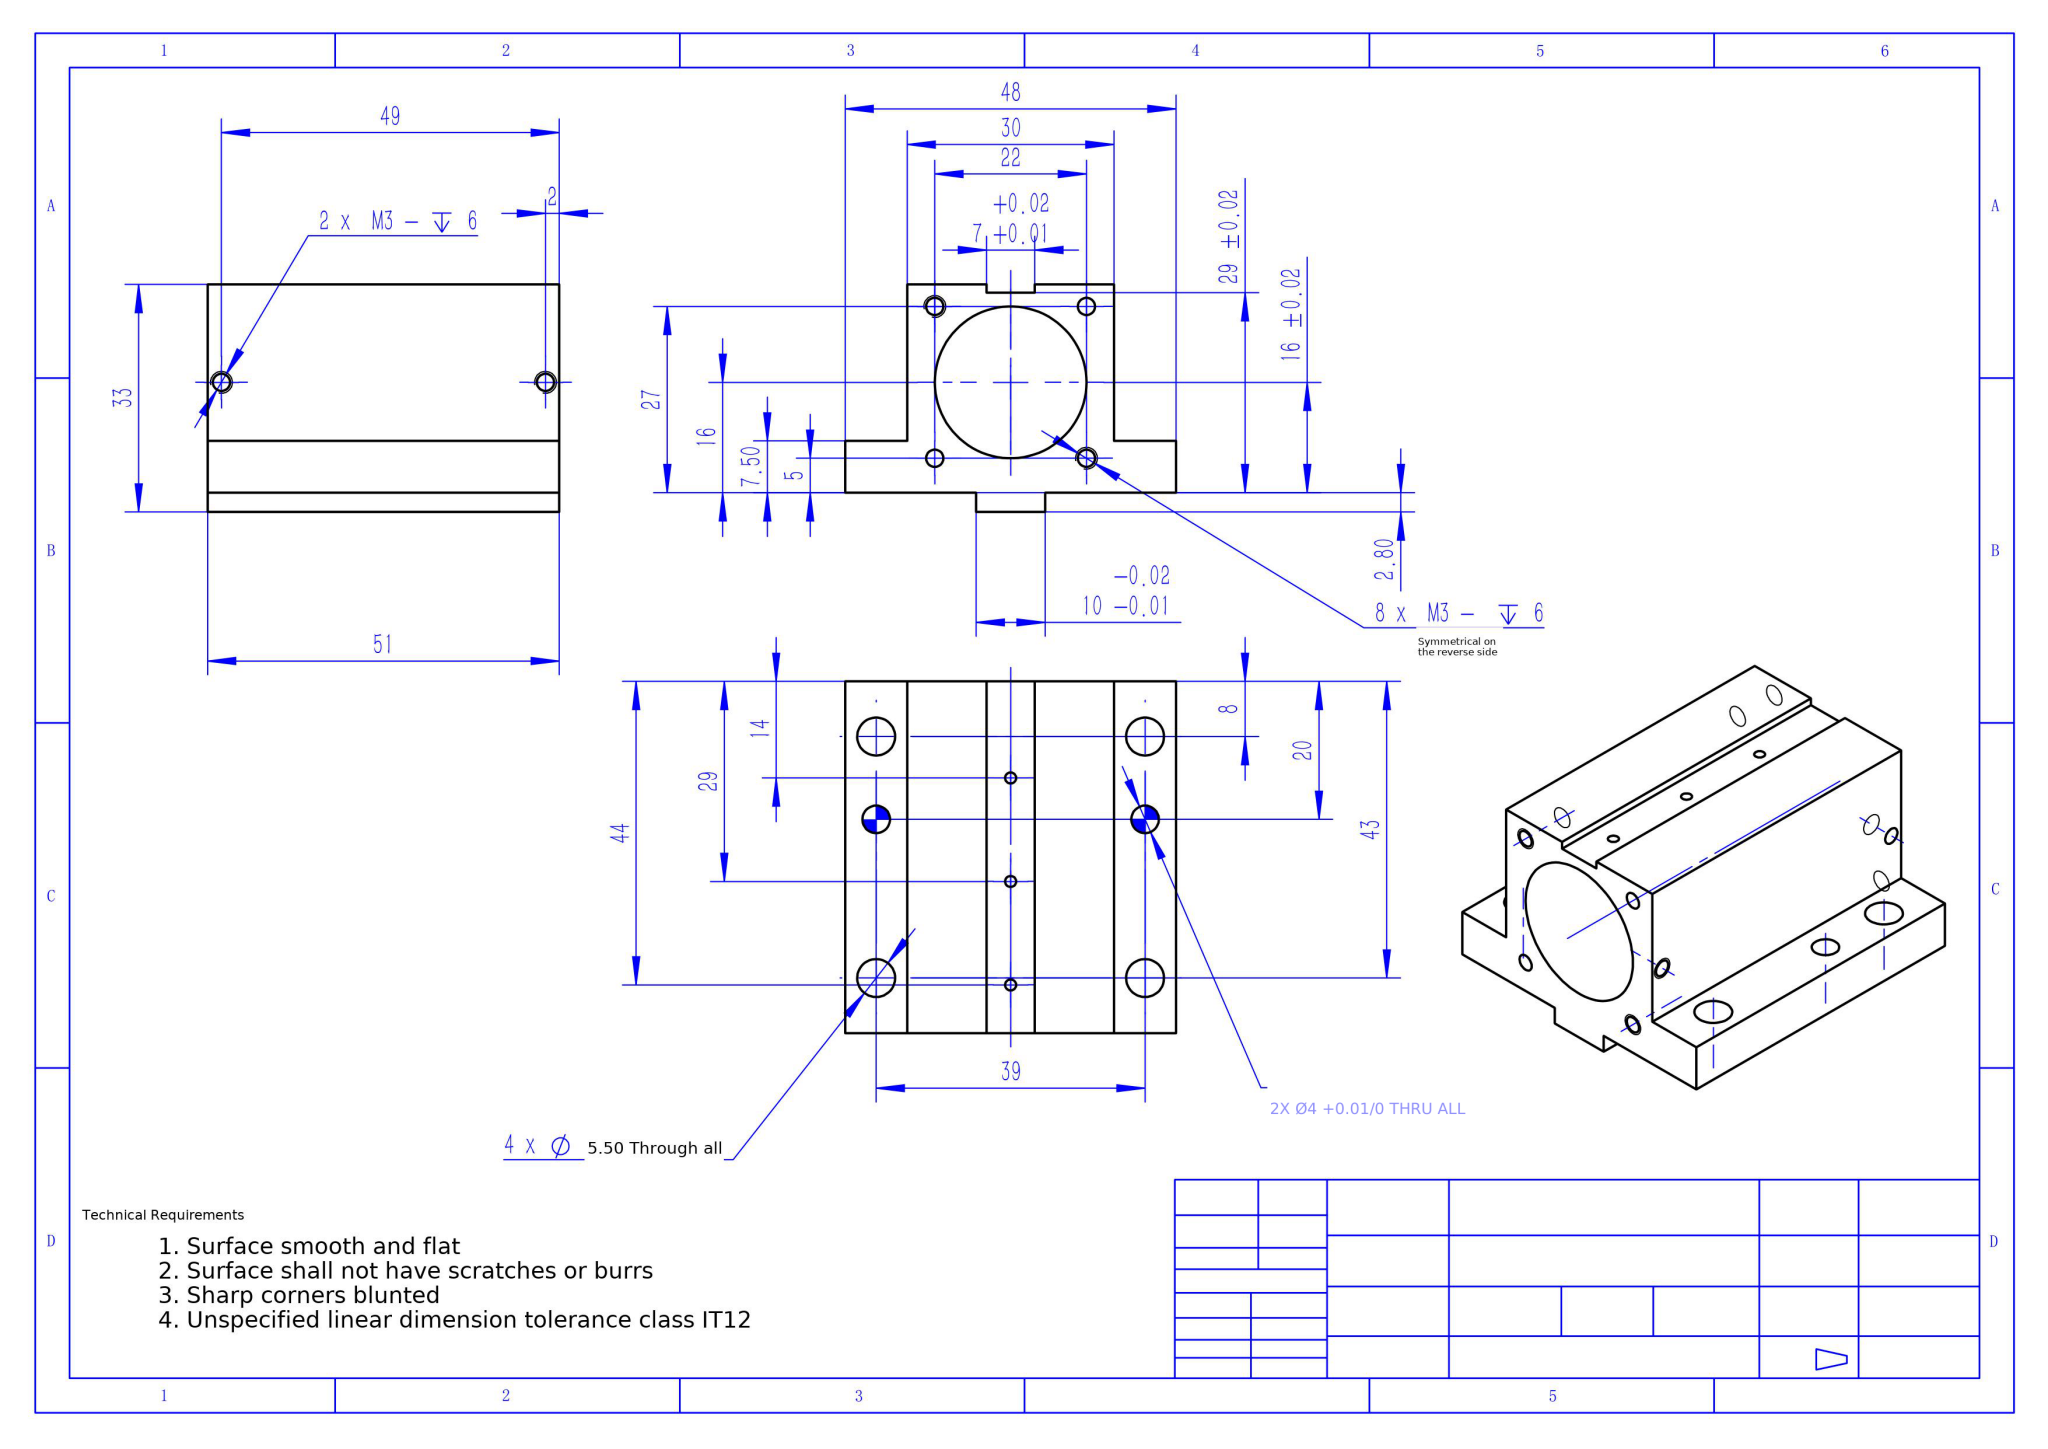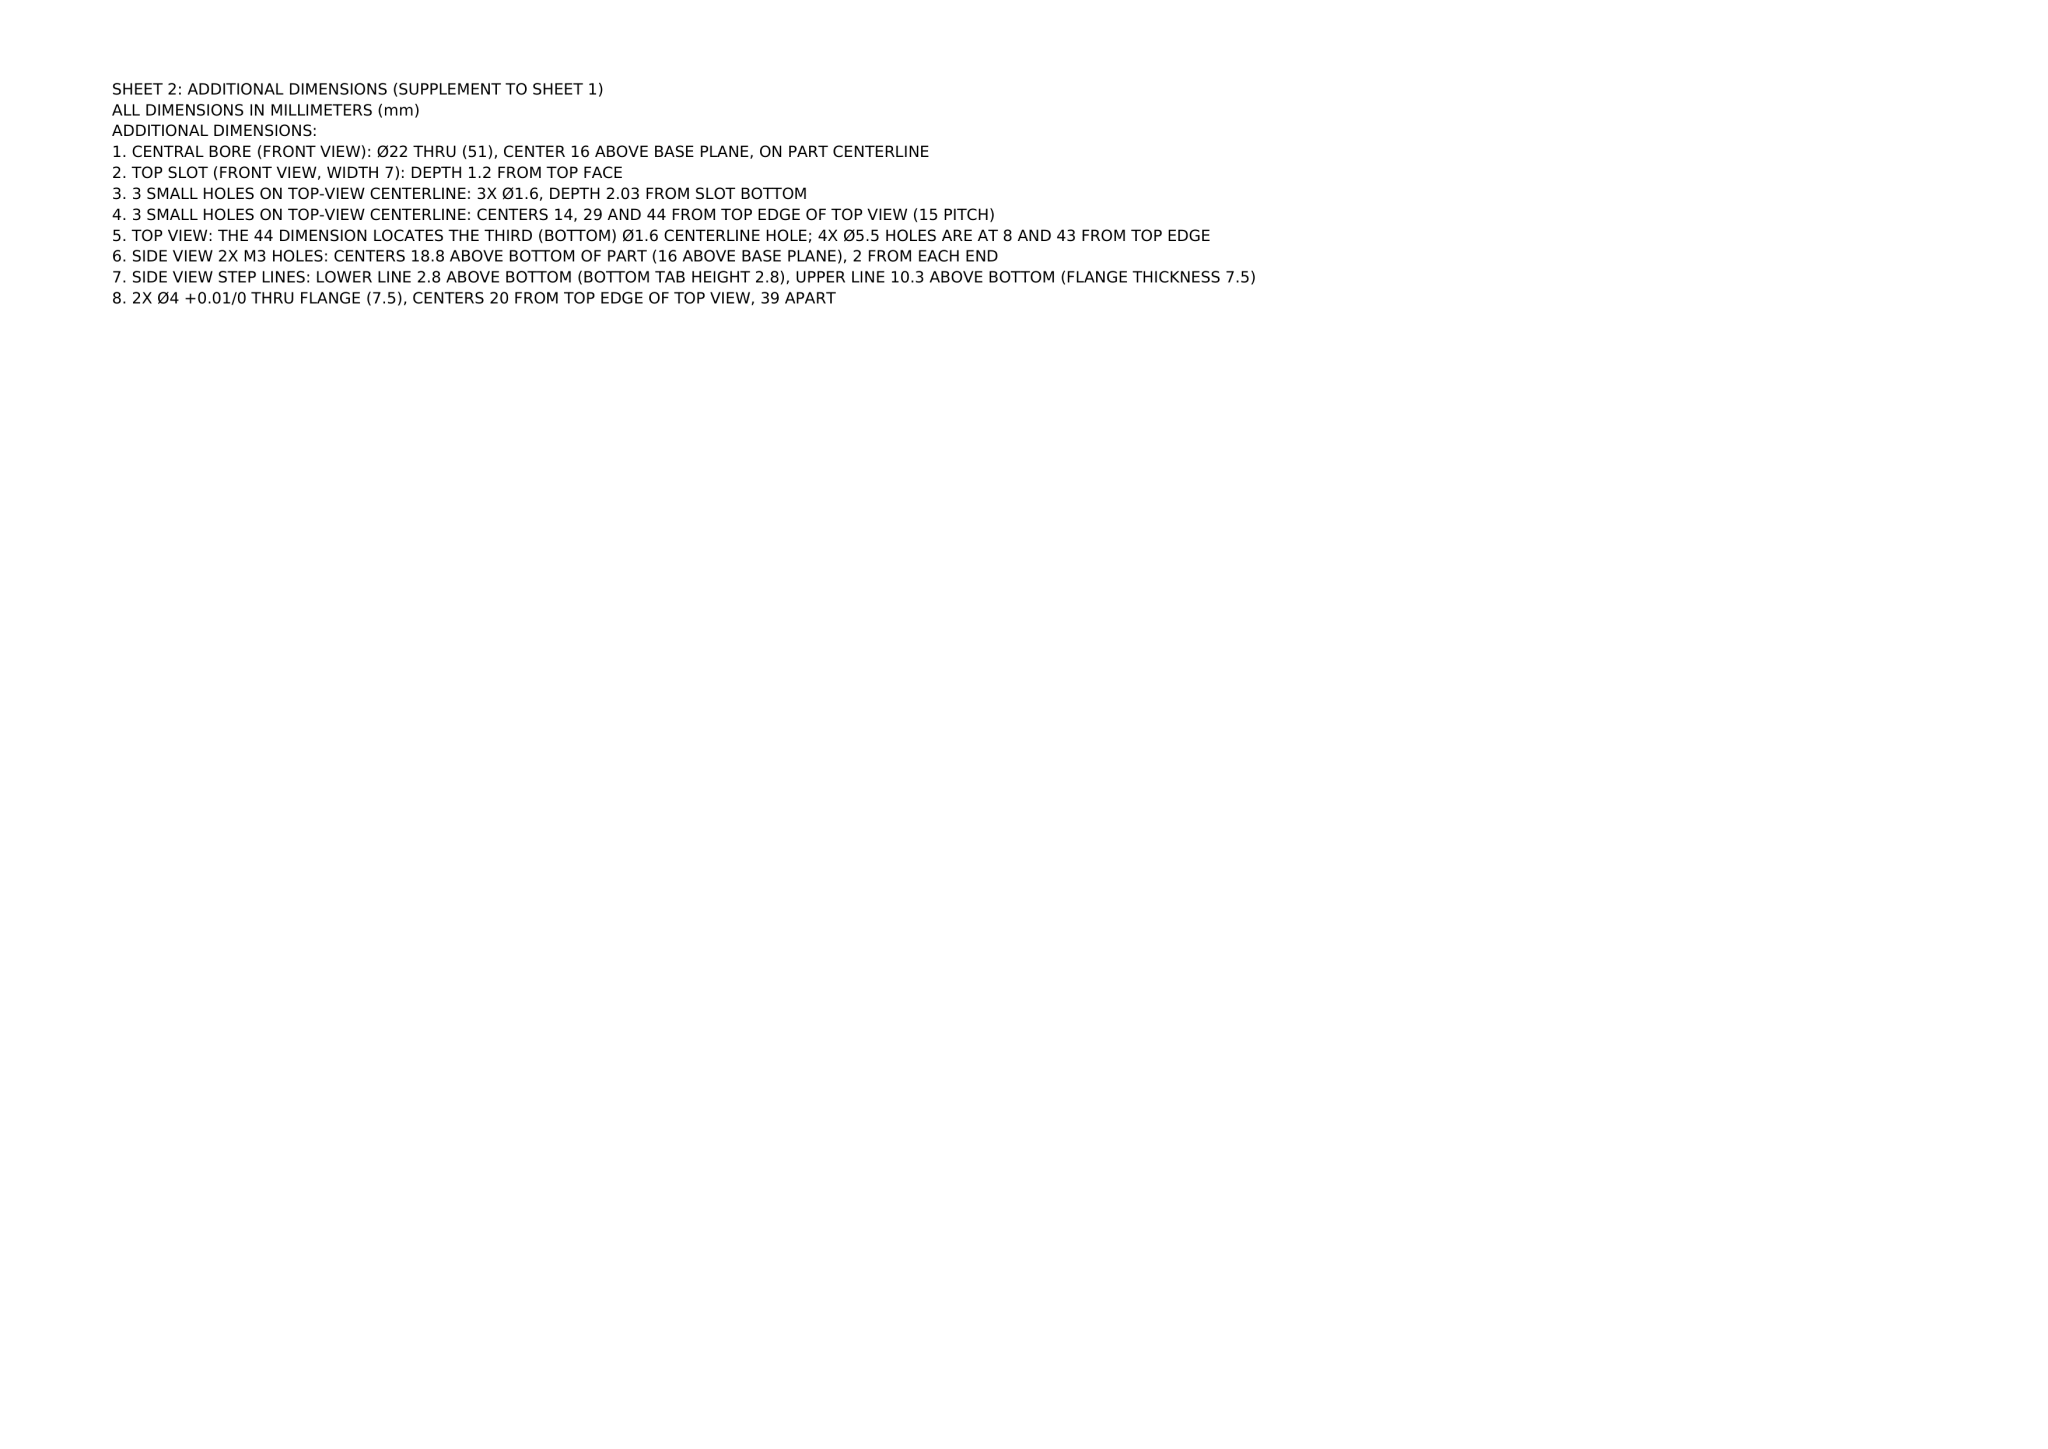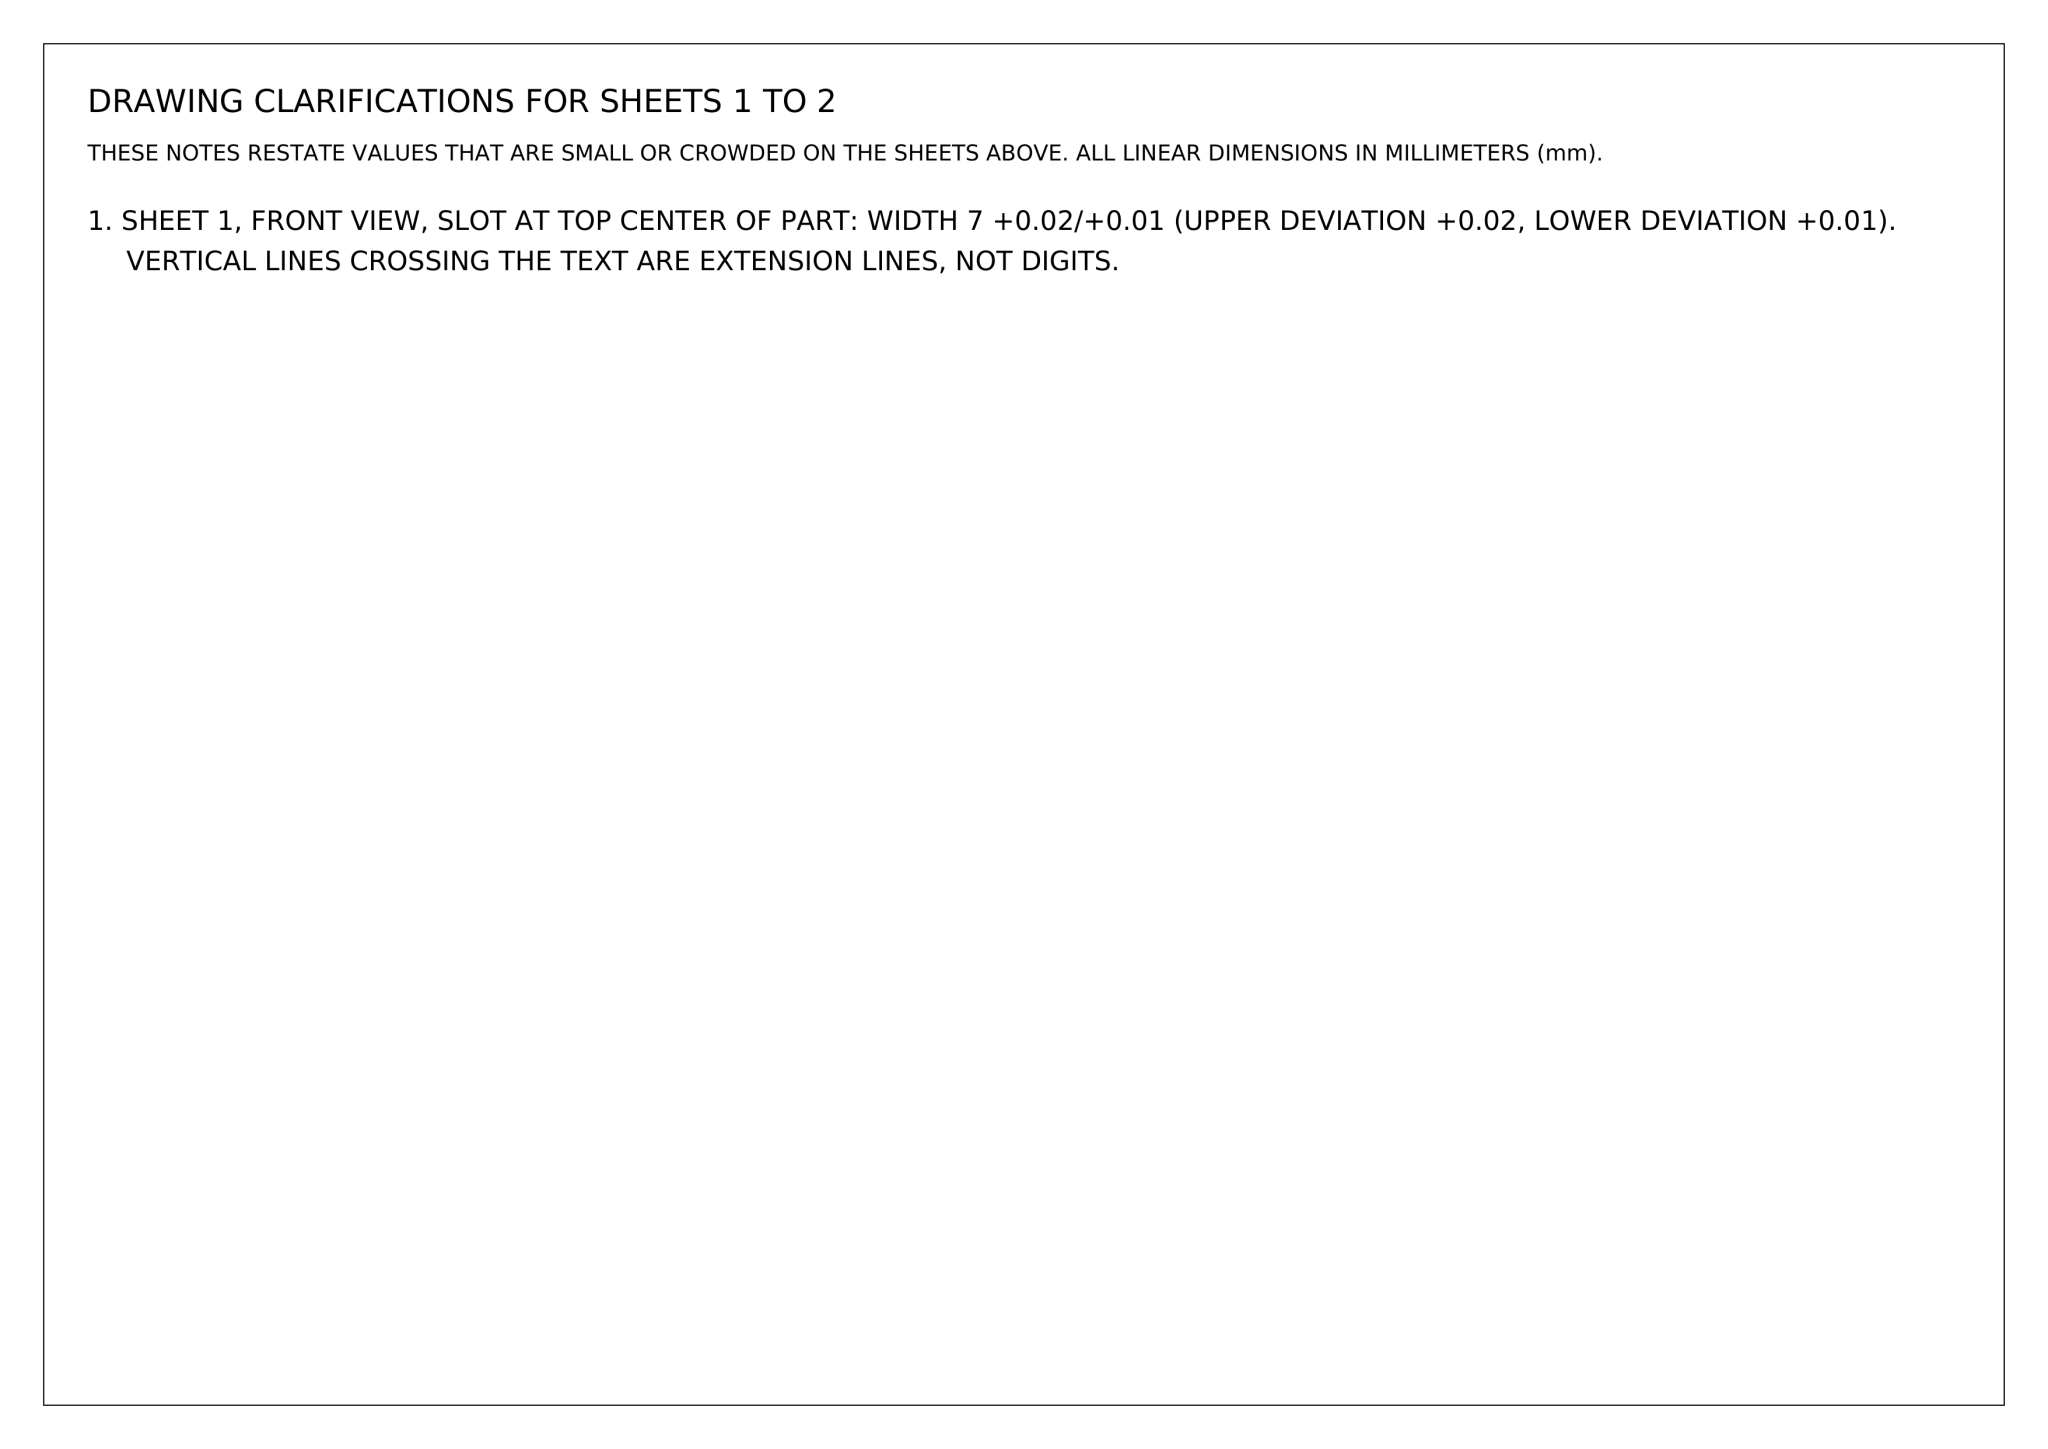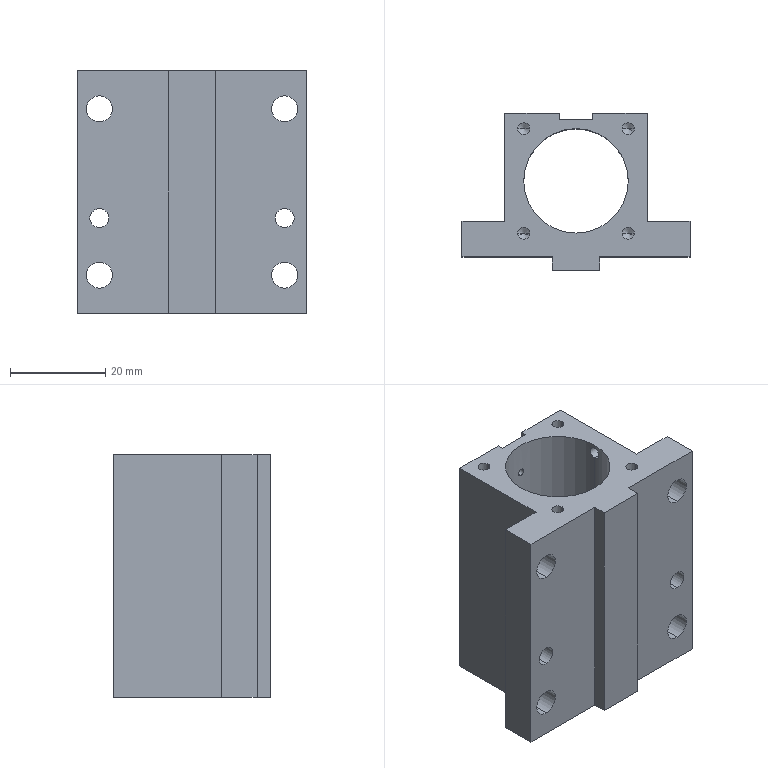Part | NX | mm | 1 solid | 74 faces | box 48 x 33 x 51 mm | volume 33447 mm3 | cylinder 40 | plane 18 | cone 16 | commonest cylinder face diameters 2.5 x20 5.5 x8 1.6 x6 4 x4 22 x2